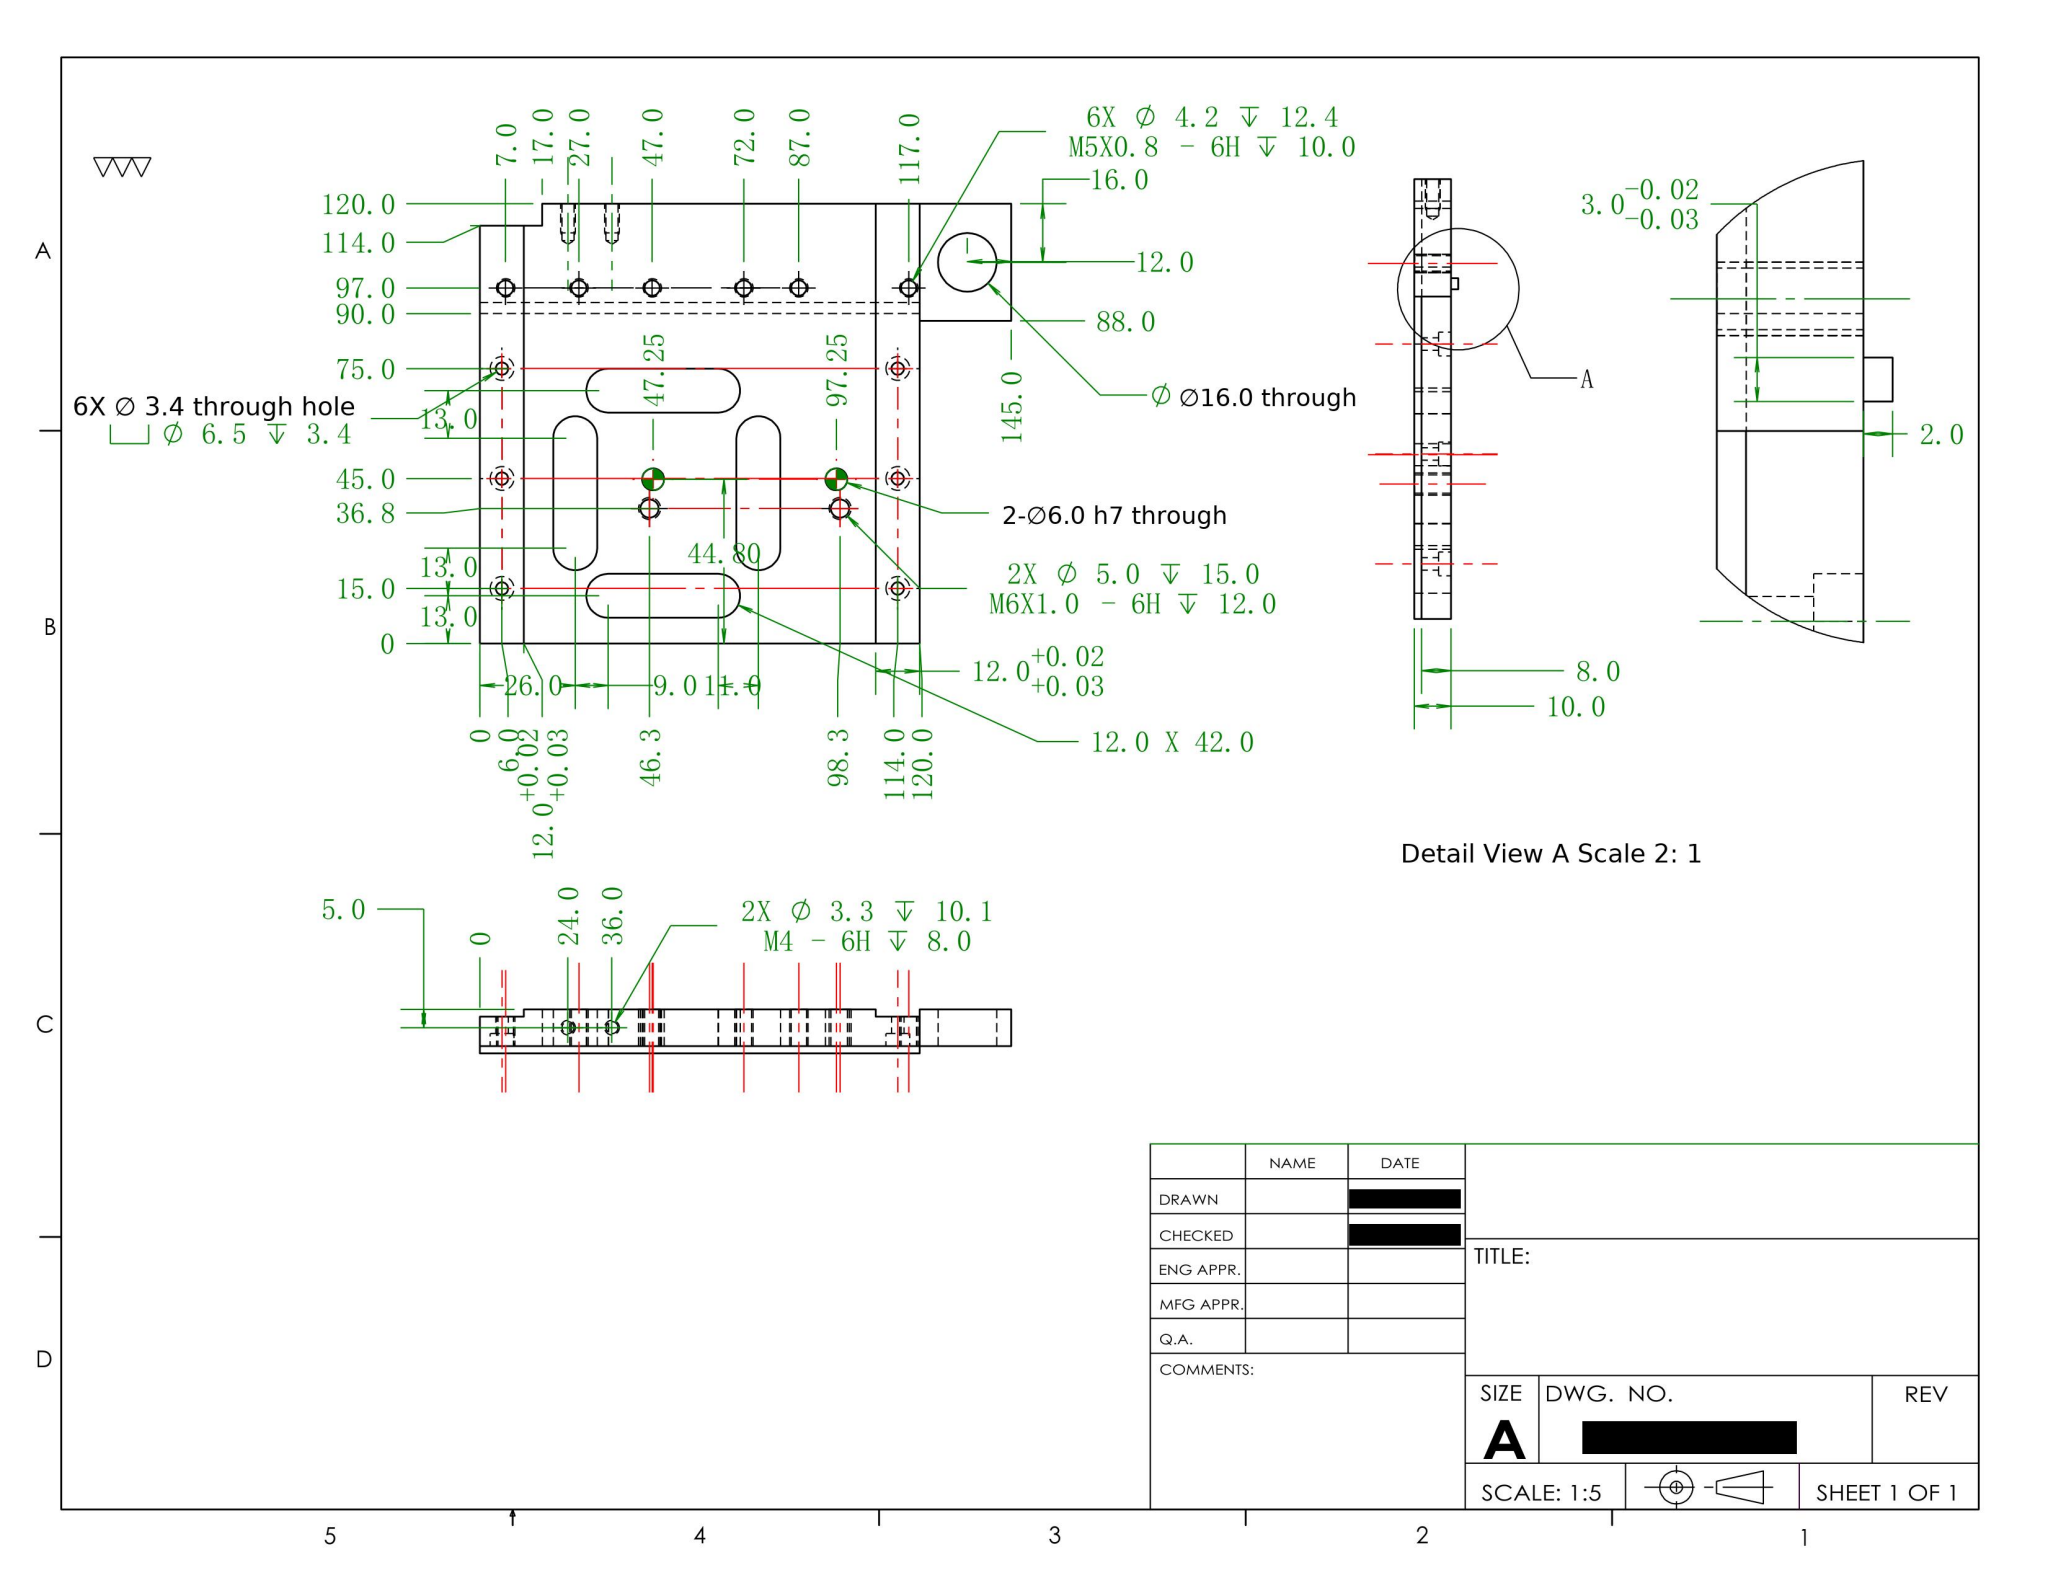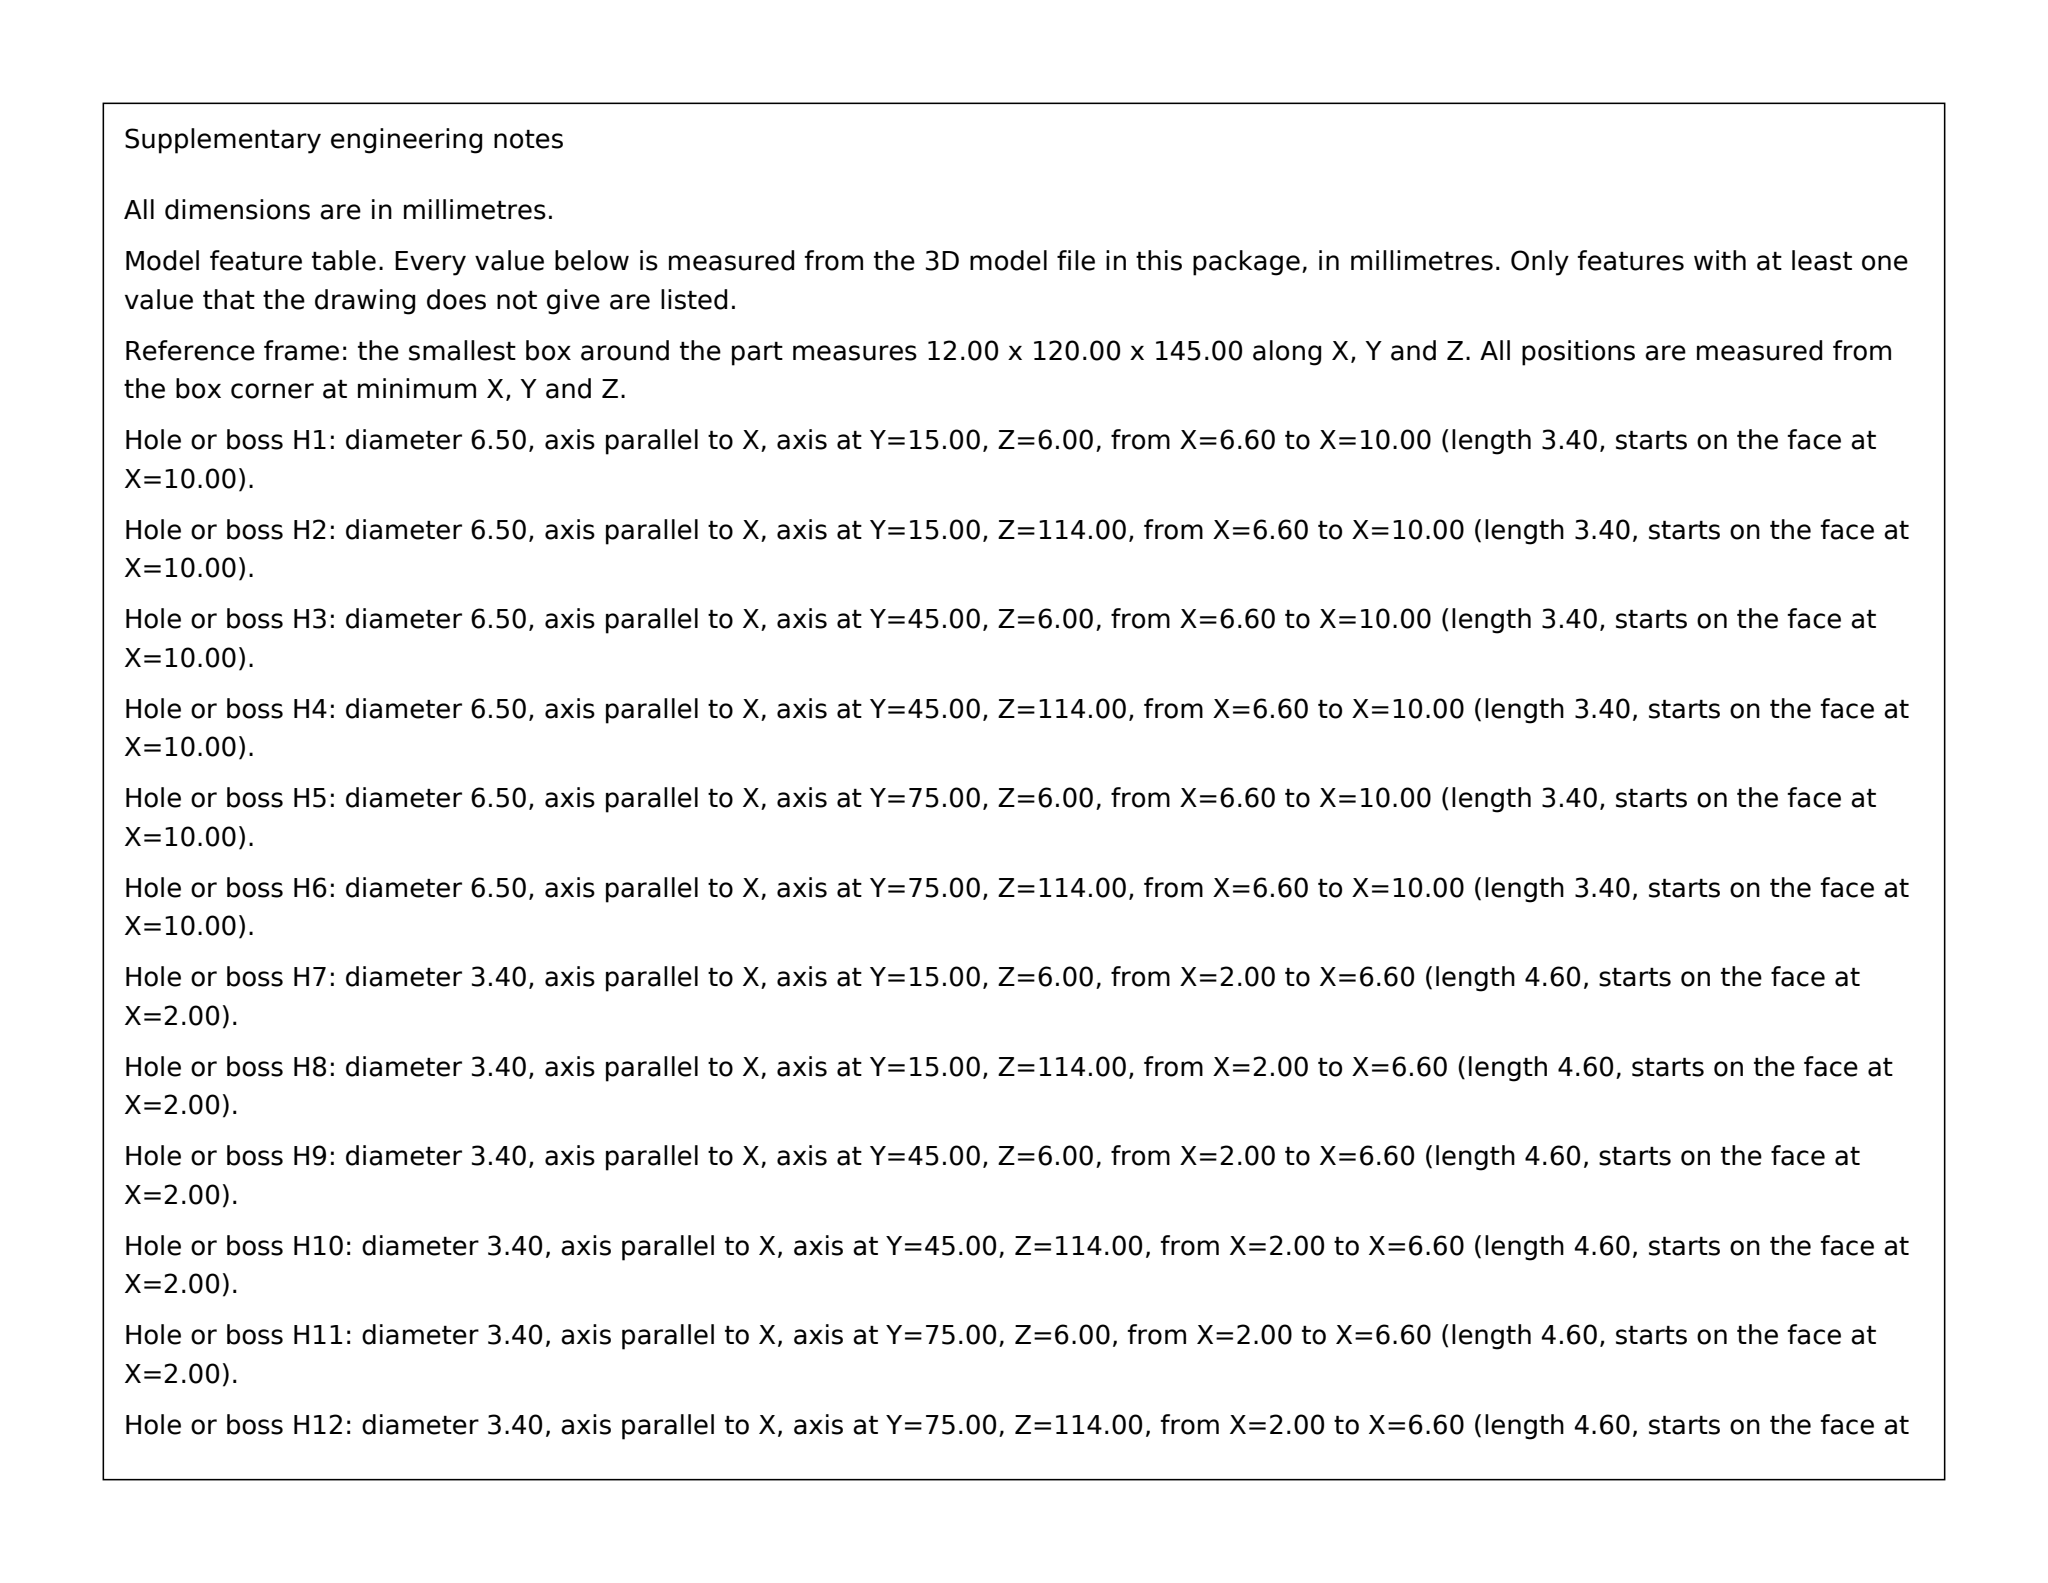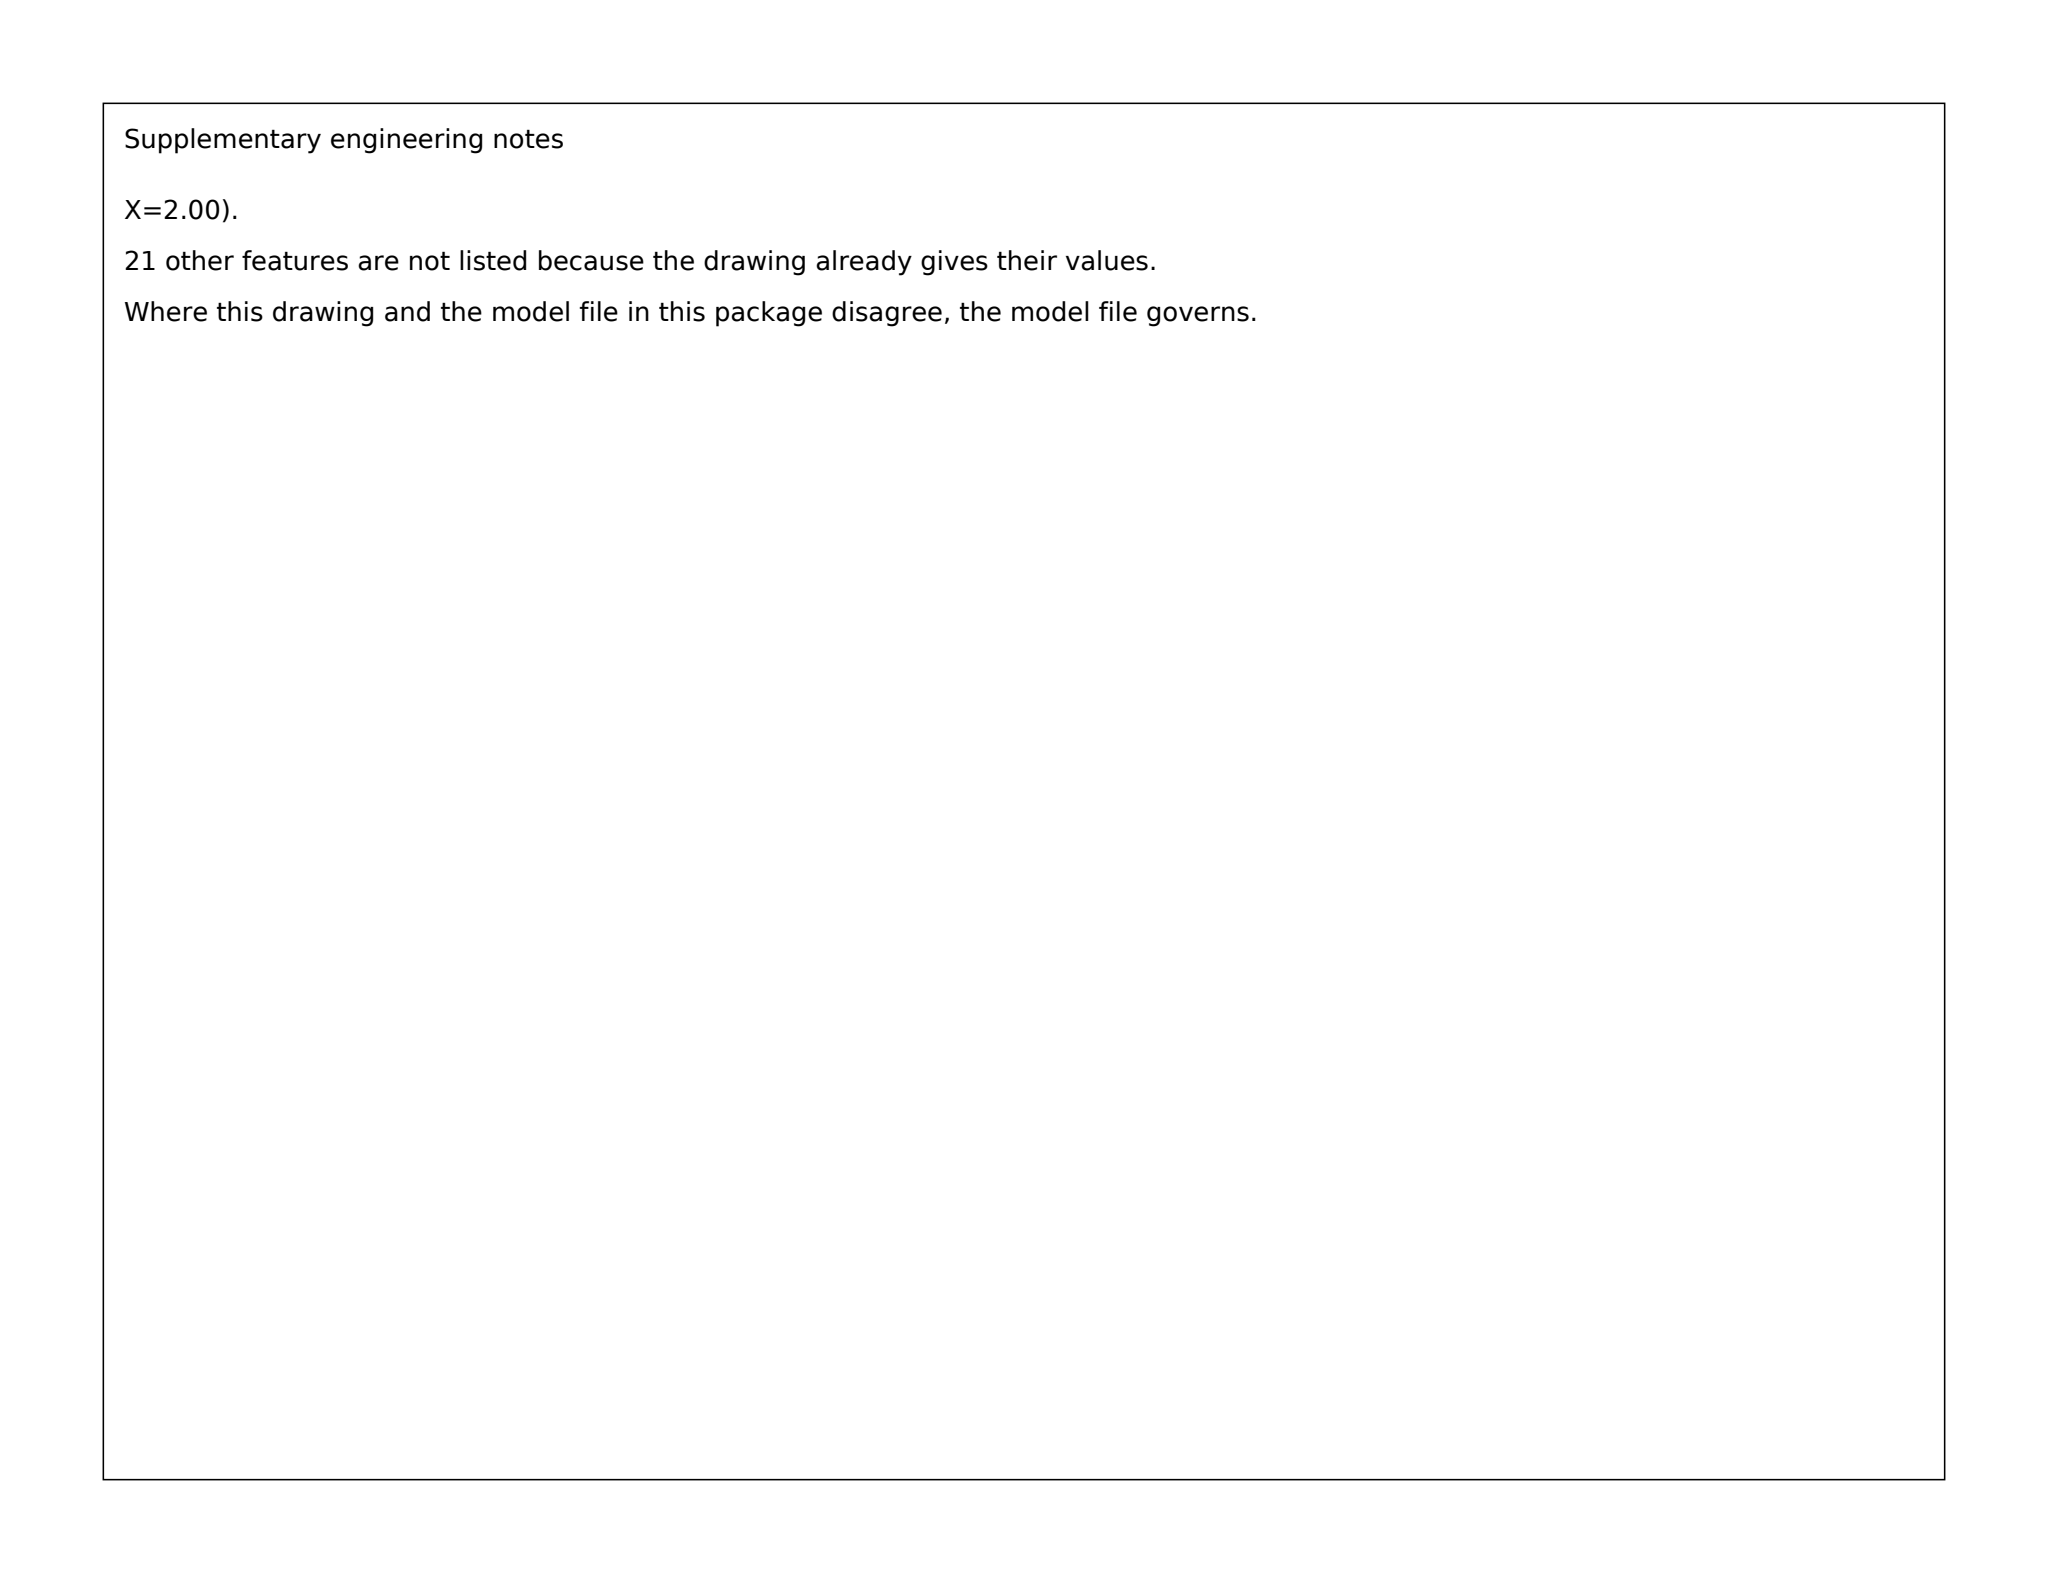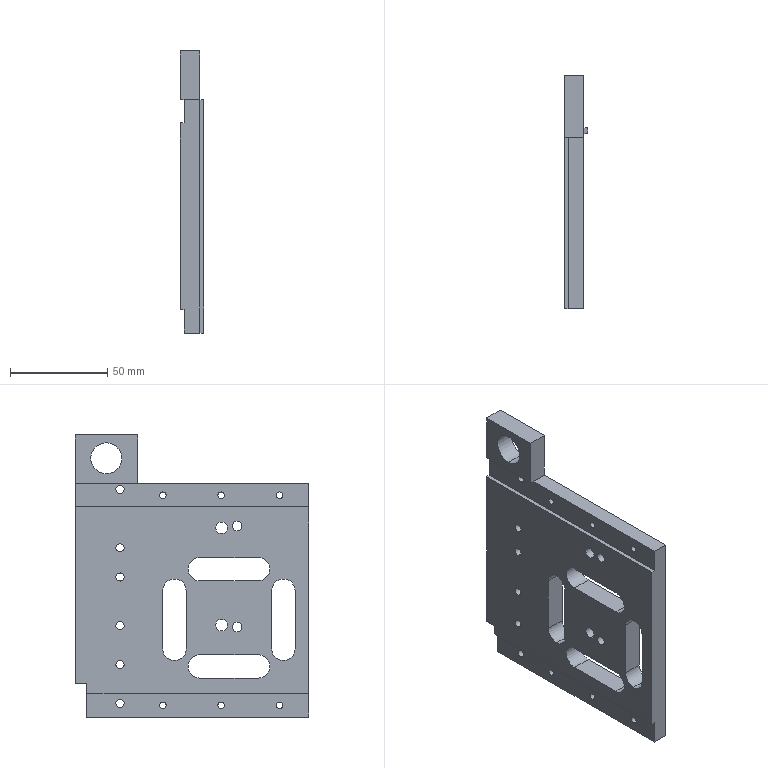Part | SolidWorks | mm | 1 solid | 98 faces | box 12 x 120 x 145 mm | volume 122310 mm3 | cylinder 60 | plane 34 | cone 4 | commonest cylinder face diameters 3.4 x12 6.5 x12 4.2 x12 12 x10 3.3 x4 6 x4 5 x4 16 x2
build123d program:
from build123d import *

# Parameters (mm, degrees)
SKETCH1_W                                       = 120
SKETCH1_H                                       = 80
EXTRUDE1_DEPTH                                  = 10
SKETCH2_W                                       = 120
SKETCH2_H                                       = 3
EXTRUDE2_DEPTH                                  = 2
LPATTERN1_COUNT                                 = 3
LPATTERN1_PITCH                                 = 40
SKETCH9_W                                       = 10
SKETCH9_H                                       = 22
EXTRUDE7_DEPTH                                  = 10
SKETCH10_W                                      = 10
SKETCH10_H                                      = 22
EXTRUDE8_DEPTH                                  = 15
SKETCH11_W                                      = 12
SKETCH11_H                                      = 80
EXTRUDE9_DEPTH                                  = 2
EXTRUDE10_DEPTH                                 = 40
EXTRUDE12_DEPTH                                 = 10
M6X1_0_TAPPED_HOLE1_D                           = 5
M6X1_0_TAPPED_HOLE1_DEPTH                       = 15
M6X1_0_TAPPED_HOLE1_TIP                         = 1.502
SKETCH17_R                                      = 3
CUT_EXTRUDE1_DEPTH                              = 145.568
M5X0_8_TAPPED_HOLE2_D                           = 4.2
M5X0_8_TAPPED_HOLE2_DEPTH                       = 12.4
M5X0_8_TAPPED_HOLE2_TIP                         = 1.262
M3_HEX_SOCKET_HEAD_CAP_SCREW_CBORE1_D           = 3.4
M3_HEX_SOCKET_HEAD_CAP_SCREW_CBORE1_CBORE_D     = 6.5
M3_HEX_SOCKET_HEAD_CAP_SCREW_CBORE1_CBORE_DEPTH = 3.4
LPATTERN2_COUNT                                 = 3
LPATTERN2_PITCH                                 = 30
SKETCH22_W                                      = 17
SKETCH22_H                                      = 6
CUT_EXTRUDE2_DEPTH                              = 10
M4_TAPPED_HOLE1_D                               = 3.3
M4_TAPPED_HOLE1_DEPTH                           = 10.1
M4_TAPPED_HOLE1_TIP                             = 0.9914
CUT_EXTRUDE3_DEPTH                              = 10
SKETCH26_R                                      = 8
CUT_EXTRUDE6_DEPTH                              = 145.568


with BuildPart() as part:
    # Sketch1 → Extrude1 (new body)
    with BuildSketch(Plane(origin=(0, 0, 0), x_dir=(0, 0, -1), z_dir=(1, 0, 0))):
        with Locations((60, 40)):
            Rectangle(SKETCH1_W, SKETCH1_H)
    extrude(amount=EXTRUDE1_DEPTH)

    # Sketch2 → Extrude2 (add)
    with BuildSketch(Plane(origin=(10, 0, 0), x_dir=(0, 0, -1), z_dir=(1, 0, 0))):
        with Locations((60, 51.5)):
            Rectangle(SKETCH2_W, SKETCH2_H)
    extrude(amount=EXTRUDE2_DEPTH)

    # Sketch3 → M5x0.8 Tapped Hole1 (revolve, cut)
    with BuildSketch(Plane(origin=(10, 57, -33), x_dir=(0, 0, -1), z_dir=(0, 1, 0))):
        Polygon((0, 0), (0, 13.662), (2.1, 12.4), (2.1, 0), align=None)
    m5x0_8_tapped_hole1 = revolve(axis=Axis((16.35, 57, -33), (-1, 0, 0)), mode=Mode.SUBTRACT)

    # LPattern1: M5x0.8 Tapped Hole1 ×3
    with Locations(*[(0, 0, -i * LPATTERN1_PITCH) for i in range(1, LPATTERN1_COUNT)]):
        add(m5x0_8_tapped_hole1, mode=Mode.SUBTRACT)

    # Sketch9 → Extrude7 (add)
    with BuildSketch(Plane.XY):
        with Locations((5, 69)):
            Rectangle(SKETCH9_W, SKETCH9_H)
    extrude(amount=EXTRUDE7_DEPTH)

    # Sketch10 → Extrude8 (add)
    with BuildSketch(Plane.XY.offset(10)):
        with Locations((5, 69)):
            Rectangle(SKETCH10_W, SKETCH10_H)
    extrude(amount=EXTRUDE8_DEPTH)

    # Sketch11 → Extrude9 (cut)
    with BuildSketch(Plane.ZY):
        with Locations((-114, 40)):
            Rectangle(SKETCH11_W, SKETCH11_H)
        with Locations((-6, 40)):
            Rectangle(SKETCH11_W, SKETCH11_H)
    extrude(amount=-EXTRUDE9_DEPTH, mode=Mode.SUBTRACT)

    # Sketch12 → Extrude10 (add)
    with BuildSketch(Plane.XZ):
        Polygon((2, 0), (2, -12), (0, -12), (0, -108), (2, -108), (2, -120), (10, -120), (10, 0), align=None)
    extrude(amount=EXTRUDE10_DEPTH)

    # Sketch14 → Extrude12 (add)
    with BuildSketch(Plane.XZ.offset(-58)):
        Polygon((0, 0), (2, 0), (10, 0), (10, 25), (0, 25), align=None)
    extrude(amount=EXTRUDE12_DEPTH)

    # M6x1.0 Tapped Hole1
    with Locations(Plane(origin=(10, 0, 0), x_dir=(0, 0, -1), z_dir=(1, 0, 0))):
        with Locations((21.75, -3.2), (73.75, -3.2)):
            Hole(M6X1_0_TAPPED_HOLE1_D / 2, depth=M6X1_0_TAPPED_HOLE1_DEPTH)
            with Locations((0, 0, -(M6X1_0_TAPPED_HOLE1_DEPTH + M6X1_0_TAPPED_HOLE1_TIP / 2))):  # 118° drill point
                Cone(0, M6X1_0_TAPPED_HOLE1_D / 2, M6X1_0_TAPPED_HOLE1_TIP, mode=Mode.SUBTRACT)

    # Sketch17 → Cut-Extrude1 (cut, through all)
    with BuildSketch(Plane(origin=(10, 0, 0), x_dir=(0, 0, -1), z_dir=(1, 0, 0))):
        with Locations((22.75, 4.8)):
            Circle(SKETCH17_R)
        with Locations((72.75, 4.8)):
            Circle(SKETCH17_R)
    extrude(amount=-CUT_EXTRUDE1_DEPTH, mode=Mode.SUBTRACT)

    # M5x0.8 Tapped Hole2
    with Locations(Plane(origin=(10, 0, 0), x_dir=(0, 0, -1), z_dir=(1, 0, 0))):
        with Locations((3, 57), (48, 57), (93, 57)):
            Hole(M5X0_8_TAPPED_HOLE2_D / 2, depth=M5X0_8_TAPPED_HOLE2_DEPTH)
            with Locations((0, 0, -(M5X0_8_TAPPED_HOLE2_DEPTH + M5X0_8_TAPPED_HOLE2_TIP / 2))):  # 118° drill point
                Cone(0, M5X0_8_TAPPED_HOLE2_D / 2, M5X0_8_TAPPED_HOLE2_TIP, mode=Mode.SUBTRACT)

    # M3 Hex Socket Head Cap Screw CBORE1 (through all)
    with Locations(Plane(origin=(10, 0, 0), x_dir=(0, 0, -1), z_dir=(1, 0, 0))):
        with Locations((6, -25), (114, -25)):
            m3_hex_socket_head_cap_screw_cbore1 = CounterBoreHole(M3_HEX_SOCKET_HEAD_CAP_SCREW_CBORE1_D / 2, M3_HEX_SOCKET_HEAD_CAP_SCREW_CBORE1_CBORE_D / 2, M3_HEX_SOCKET_HEAD_CAP_SCREW_CBORE1_CBORE_DEPTH)

    # LPattern2: M3 Hex Socket Head Cap Screw CBORE1 ×3
    with Locations(*[(0, i * LPATTERN2_PITCH, 0) for i in range(1, LPATTERN2_COUNT)]):
        add(m3_hex_socket_head_cap_screw_cbore1, mode=Mode.SUBTRACT)

    # Sketch22 → Cut-Extrude2 (cut)
    with BuildSketch(Plane(origin=(10, 0, 0), x_dir=(0, 0, -1), z_dir=(1, 0, 0))):
        with Locations((111.5, 77)):
            Rectangle(SKETCH22_W, SKETCH22_H)
    extrude(amount=-CUT_EXTRUDE2_DEPTH, mode=Mode.SUBTRACT)

    # M4 Tapped Hole1
    with Locations(Plane(origin=(0, 80, 0), x_dir=(-1, 0, 0), z_dir=(0, 1, 0))):
        with Locations((-5, -96), (-5, -84)):
            Hole(M4_TAPPED_HOLE1_D / 2, depth=M4_TAPPED_HOLE1_DEPTH)
            with Locations((0, 0, -(M4_TAPPED_HOLE1_DEPTH + M4_TAPPED_HOLE1_TIP / 2))):  # 118° drill point
                Cone(0, M4_TAPPED_HOLE1_D / 2, M4_TAPPED_HOLE1_TIP, mode=Mode.SUBTRACT)

    # Sketch25 → Cut-Extrude3 (cut)
    with BuildSketch(Plane(origin=(10, 0, 0), x_dir=(0, 0, -1), z_dir=(1, 0, 0))):
        with BuildLine():
            Line((50, 16), (50, -14))
            ThreePointArc((50, -14), (44, -20), (38, -14))
            Line((38, -14), (38, 16))
            ThreePointArc((38, 16), (44, 22), (50, 16))
        make_face()
        with BuildLine():
            Line((100, 16), (100, -14))
            ThreePointArc((100, -14), (94, -20), (88, -14))
            Line((88, -14), (88, 16))
            ThreePointArc((88, 16), (94, 22), (100, 16))
        make_face()
        with BuildLine():
            Line((55, 35), (85, 35))
            ThreePointArc((85, 35), (91, 29), (85, 23))
            Line((85, 23), (55, 23))
            ThreePointArc((55, 23), (49, 29), (55, 35))
        make_face()
        with BuildLine():
            Line((55, -21), (85, -21))
            ThreePointArc((85, -21), (91, -27), (85, -33))
            Line((85, -33), (55, -33))
            ThreePointArc((55, -33), (49, -27), (55, -21))
        make_face()
    extrude(amount=-CUT_EXTRUDE3_DEPTH, mode=Mode.SUBTRACT)

    # Sketch26 → Cut-Extrude6 (cut, through all)
    with BuildSketch(Plane(origin=(10, 0, 0), x_dir=(0, 0, -1), z_dir=(1, 0, 0))):
        with Locations((-13, 64)):
            Circle(SKETCH26_R)
    extrude(amount=-CUT_EXTRUDE6_DEPTH, mode=Mode.SUBTRACT)


solid = part.part